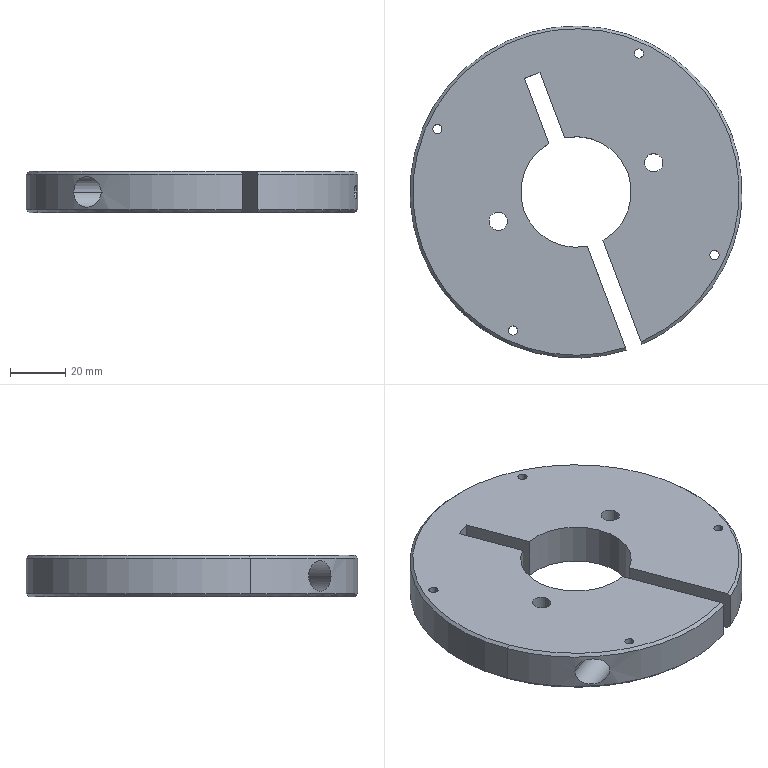Component | SolidWorks | 8TC-A17001-20-03LocatingPlate-1 | 1 solid | 44 faces | volume 137677 mm3 | cylinder 28 | plane 10 | cone 6 | commonest cylinder face diameters 3.3 x8 11 x6 6.6 x6 120 x3 40 x3 5 x2 | material 6061 Alloy